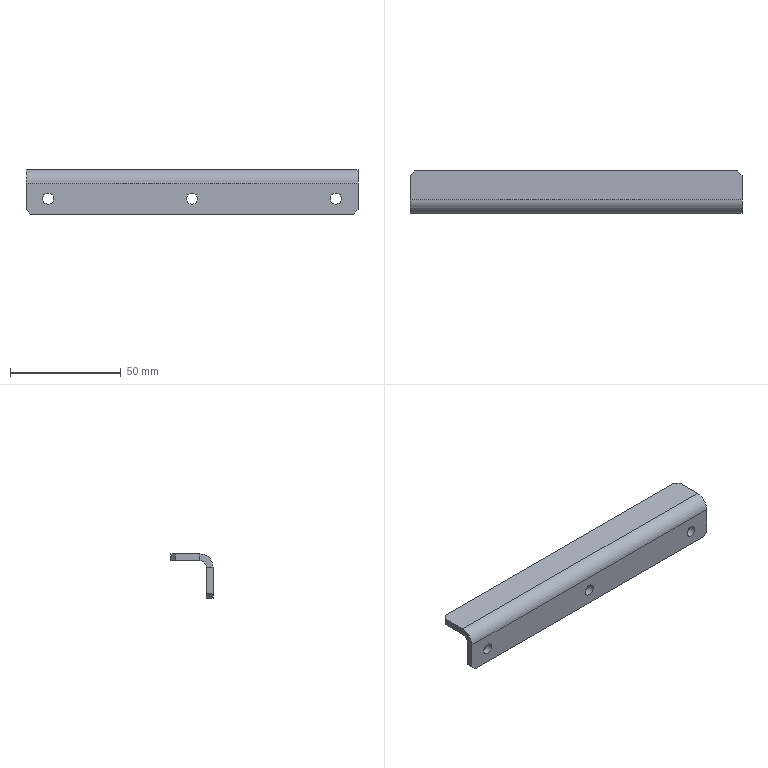Component | SolidWorks | MTCTV2104DJ006-000-0002PressurePlate-1 | 1 solid | 24 faces | box 150 x 19 x 20 mm | volume 15130 mm3 | plane 16 | cylinder 8 | commonest cylinder face diameters 5 x6 12 x1 6 x1
STEP:
#1=CARTESIAN_POINT('',(-7.285,3.002,8.574));
#2=VERTEX_POINT('',#1);
#3=CARTESIAN_POINT('',(-7.482,3.002,8.574));
#4=VERTEX_POINT('',#3);
#5=CARTESIAN_POINT('',(-7.383,3.002,8.574));
#6=DIRECTION('',(-0.,1.,0.));
#7=DIRECTION('',(-1.,0.,0.));
#8=AXIS2_PLACEMENT_3D('',#5,#6,#7);
#9=CIRCLE('',#8,0.09843);
#10=EDGE_CURVE('',#2,#4,#9,.T.);
#11=ORIENTED_EDGE('',*,*,#10,.T.);
#12=CARTESIAN_POINT('',(-7.482,2.884,8.574));
#13=VERTEX_POINT('',#12);
#14=CARTESIAN_POINT('',(-7.482,2.884,8.574));
#15=DIRECTION('',(0.,-1.,-0.));
#16=VECTOR('',#15,39.37);
#17=LINE('',#14,#16);
#18=EDGE_CURVE('',#4,#13,#17,.T.);
#19=ORIENTED_EDGE('',*,*,#18,.T.);
#20=CARTESIAN_POINT('',(-7.285,2.884,8.574));
#21=VERTEX_POINT('',#20);
#22=CARTESIAN_POINT('',(-7.383,2.884,8.574));
#23=DIRECTION('',(0.,-1.,-0.));
#24=DIRECTION('',(1.,0.,0.));
#25=AXIS2_PLACEMENT_3D('',#22,#23,#24);
#26=CIRCLE('',#25,0.09843);
#27=EDGE_CURVE('',#13,#21,#26,.T.);
#28=ORIENTED_EDGE('',*,*,#27,.T.);
#29=CARTESIAN_POINT('',(-7.285,2.884,8.574));
#30=DIRECTION('',(0.,-1.,-0.));
#31=VECTOR('',#30,39.37);
#32=LINE('',#29,#31);
#33=EDGE_CURVE('',#2,#21,#32,.T.);
#34=ORIENTED_EDGE('',*,*,#33,.F.);
#35=EDGE_LOOP('',(#11,#19,#28,#34));
#36=FACE_OUTER_BOUND('',#35,.T.);
#37=CARTESIAN_POINT('',(-7.383,2.884,8.574));
#38=DIRECTION('',(0.,-1.,-0.));
#39=DIRECTION('',(1.,0.,0.));
#40=AXIS2_PLACEMENT_3D('',#37,#38,#39);
#41=CYLINDRICAL_SURFACE('',#40,0.09843);
#42=ADVANCED_FACE('',(#36),#41,.F.);
#43=CARTESIAN_POINT('',(-4.726,3.002,8.574));
#44=VERTEX_POINT('',#43);
#45=CARTESIAN_POINT('',(-4.923,3.002,8.574));
#46=VERTEX_POINT('',#45);
#47=CARTESIAN_POINT('',(-4.824,3.002,8.574));
#48=DIRECTION('',(-0.,1.,0.));
#49=DIRECTION('',(-1.,0.,0.));
#50=AXIS2_PLACEMENT_3D('',#47,#48,#49);
#51=CIRCLE('',#50,0.09843);
#52=EDGE_CURVE('',#44,#46,#51,.T.);
#53=ORIENTED_EDGE('',*,*,#52,.T.);
#54=CARTESIAN_POINT('',(-4.923,2.884,8.574));
#55=VERTEX_POINT('',#54);
#56=CARTESIAN_POINT('',(-4.923,2.884,8.574));
#57=DIRECTION('',(0.,-1.,-0.));
#58=VECTOR('',#57,39.37);
#59=LINE('',#56,#58);
#60=EDGE_CURVE('',#46,#55,#59,.T.);
#61=ORIENTED_EDGE('',*,*,#60,.T.);
#62=CARTESIAN_POINT('',(-4.726,2.884,8.574));
#63=VERTEX_POINT('',#62);
#64=CARTESIAN_POINT('',(-4.824,2.884,8.574));
#65=DIRECTION('',(0.,-1.,-0.));
#66=DIRECTION('',(1.,0.,0.));
#67=AXIS2_PLACEMENT_3D('',#64,#65,#66);
#68=CIRCLE('',#67,0.09843);
#69=EDGE_CURVE('',#55,#63,#68,.T.);
#70=ORIENTED_EDGE('',*,*,#69,.T.);
#71=CARTESIAN_POINT('',(-4.726,2.884,8.574));
#72=DIRECTION('',(0.,-1.,-0.));
#73=VECTOR('',#72,39.37);
#74=LINE('',#71,#73);
#75=EDGE_CURVE('',#44,#63,#74,.T.);
#76=ORIENTED_EDGE('',*,*,#75,.F.);
#77=EDGE_LOOP('',(#53,#61,#70,#76));
#78=FACE_OUTER_BOUND('',#77,.T.);
#79=CARTESIAN_POINT('',(-4.824,2.884,8.574));
#80=DIRECTION('',(0.,-1.,-0.));
#81=DIRECTION('',(1.,0.,0.));
#82=AXIS2_PLACEMENT_3D('',#79,#80,#81);
#83=CYLINDRICAL_SURFACE('',#82,0.09843);
#84=ADVANCED_FACE('',(#78),#83,.F.);
#85=CARTESIAN_POINT('',(-2.167,3.002,8.574));
#86=VERTEX_POINT('',#85);
#87=CARTESIAN_POINT('',(-2.364,3.002,8.574));
#88=VERTEX_POINT('',#87);
#89=CARTESIAN_POINT('',(-2.265,3.002,8.574));
#90=DIRECTION('',(-0.,1.,0.));
#91=DIRECTION('',(-1.,0.,0.));
#92=AXIS2_PLACEMENT_3D('',#89,#90,#91);
#93=CIRCLE('',#92,0.09843);
#94=EDGE_CURVE('',#86,#88,#93,.T.);
#95=ORIENTED_EDGE('',*,*,#94,.T.);
#96=CARTESIAN_POINT('',(-2.364,2.884,8.574));
#97=VERTEX_POINT('',#96);
#98=CARTESIAN_POINT('',(-2.364,2.884,8.574));
#99=DIRECTION('',(0.,-1.,-0.));
#100=VECTOR('',#99,39.37);
#101=LINE('',#98,#100);
#102=EDGE_CURVE('',#88,#97,#101,.T.);
#103=ORIENTED_EDGE('',*,*,#102,.T.);
#104=CARTESIAN_POINT('',(-2.167,2.884,8.574));
#105=VERTEX_POINT('',#104);
#106=CARTESIAN_POINT('',(-2.265,2.884,8.574));
#107=DIRECTION('',(0.,-1.,-0.));
#108=DIRECTION('',(1.,0.,0.));
#109=AXIS2_PLACEMENT_3D('',#106,#107,#108);
#110=CIRCLE('',#109,0.09843);
#111=EDGE_CURVE('',#97,#105,#110,.T.);
#112=ORIENTED_EDGE('',*,*,#111,.T.);
#113=CARTESIAN_POINT('',(-2.167,2.884,8.574));
#114=DIRECTION('',(0.,-1.,-0.));
#115=VECTOR('',#114,39.37);
#116=LINE('',#113,#115);
#117=EDGE_CURVE('',#86,#105,#116,.T.);
#118=ORIENTED_EDGE('',*,*,#117,.F.);
#119=EDGE_LOOP('',(#95,#103,#112,#118));
#120=FACE_OUTER_BOUND('',#119,.T.);
#121=CARTESIAN_POINT('',(-2.265,2.884,8.574));
#122=DIRECTION('',(0.,-1.,-0.));
#123=DIRECTION('',(1.,0.,0.));
#124=AXIS2_PLACEMENT_3D('',#121,#122,#123);
#125=CYLINDRICAL_SURFACE('',#124,0.09843);
#126=ADVANCED_FACE('',(#120),#125,.F.);
#127=CARTESIAN_POINT('',(-7.383,2.884,8.574));
#128=DIRECTION('',(0.,-1.,-0.));
#129=DIRECTION('',(1.,0.,0.));
#130=AXIS2_PLACEMENT_3D('',#127,#128,#129);
#131=CIRCLE('',#130,0.09843);
#132=EDGE_CURVE('',#21,#13,#131,.T.);
#133=ORIENTED_EDGE('',*,*,#132,.F.);
#134=ORIENTED_EDGE('',*,*,#27,.F.);
#135=EDGE_LOOP('',(#133,#134));
#136=FACE_BOUND('',#135,.T.);
#137=CARTESIAN_POINT('',(-2.265,2.884,8.574));
#138=DIRECTION('',(0.,-1.,-0.));
#139=DIRECTION('',(1.,0.,0.));
#140=AXIS2_PLACEMENT_3D('',#137,#138,#139);
#141=CIRCLE('',#140,0.09843);
#142=EDGE_CURVE('',#105,#97,#141,.T.);
#143=ORIENTED_EDGE('',*,*,#142,.F.);
#144=ORIENTED_EDGE('',*,*,#111,.F.);
#145=EDGE_LOOP('',(#143,#144));
#146=FACE_BOUND('',#145,.T.);
#147=CARTESIAN_POINT('',(-7.777,2.884,8.85));
#148=VERTEX_POINT('',#147);
#149=CARTESIAN_POINT('',(-7.777,2.884,8.377));
#150=VERTEX_POINT('',#149);
#151=CARTESIAN_POINT('',(-7.777,2.884,8.299));
#152=DIRECTION('',(-0.,0.,-1.));
#153=VECTOR('',#152,39.37);
#154=LINE('',#151,#153);
#155=EDGE_CURVE('',#148,#150,#154,.T.);
#156=ORIENTED_EDGE('',*,*,#155,.T.);
#157=CARTESIAN_POINT('',(-7.698,2.884,8.299));
#158=VERTEX_POINT('',#157);
#159=CARTESIAN_POINT('',(-7.777,2.884,8.377));
#160=DIRECTION('',(0.7071,0.,-0.7071));
#161=VECTOR('',#160,39.37);
#162=LINE('',#159,#161);
#163=EDGE_CURVE('',#150,#158,#162,.T.);
#164=ORIENTED_EDGE('',*,*,#163,.T.);
#165=CARTESIAN_POINT('',(-1.95,2.884,8.299));
#166=VERTEX_POINT('',#165);
#167=CARTESIAN_POINT('',(-7.777,2.884,8.299));
#168=DIRECTION('',(1.,0.,0.));
#169=VECTOR('',#168,39.37);
#170=LINE('',#167,#169);
#171=EDGE_CURVE('',#158,#166,#170,.T.);
#172=ORIENTED_EDGE('',*,*,#171,.T.);
#173=CARTESIAN_POINT('',(-1.872,2.884,8.377));
#174=VERTEX_POINT('',#173);
#175=CARTESIAN_POINT('',(-1.95,2.884,8.299));
#176=DIRECTION('',(0.7071,-0.,0.7071));
#177=VECTOR('',#176,39.37);
#178=LINE('',#175,#177);
#179=EDGE_CURVE('',#166,#174,#178,.T.);
#180=ORIENTED_EDGE('',*,*,#179,.T.);
#181=CARTESIAN_POINT('',(-1.872,2.884,8.85));
#182=VERTEX_POINT('',#181);
#183=CARTESIAN_POINT('',(-1.872,2.884,8.299));
#184=DIRECTION('',(0.,-0.,1.));
#185=VECTOR('',#184,39.37);
#186=LINE('',#183,#185);
#187=EDGE_CURVE('',#174,#182,#186,.T.);
#188=ORIENTED_EDGE('',*,*,#187,.T.);
#189=CARTESIAN_POINT('',(-1.872,2.884,8.85));
#190=DIRECTION('',(-1.,-0.,-0.));
#191=VECTOR('',#190,39.37);
#192=LINE('',#189,#191);
#193=EDGE_CURVE('',#182,#148,#192,.T.);
#194=ORIENTED_EDGE('',*,*,#193,.T.);
#195=EDGE_LOOP('',(#156,#164,#172,#180,#188,#194));
#196=FACE_OUTER_BOUND('',#195,.T.);
#197=CARTESIAN_POINT('',(-4.824,2.884,8.574));
#198=DIRECTION('',(0.,-1.,-0.));
#199=DIRECTION('',(1.,0.,0.));
#200=AXIS2_PLACEMENT_3D('',#197,#198,#199);
#201=CIRCLE('',#200,0.09843);
#202=EDGE_CURVE('',#63,#55,#201,.T.);
#203=ORIENTED_EDGE('',*,*,#202,.F.);
#204=ORIENTED_EDGE('',*,*,#69,.F.);
#205=EDGE_LOOP('',(#203,#204));
#206=FACE_BOUND('',#205,.T.);
#207=CARTESIAN_POINT('',(-4.824,2.884,8.692));
#208=DIRECTION('',(-0.,1.,0.));
#209=DIRECTION('',(-1.,-0.,-0.));
#210=AXIS2_PLACEMENT_3D('',#207,#208,#209);
#211=PLANE('',#210);
#212=ADVANCED_FACE('',(#136,#146,#196,#206),#211,.F.);
#213=ORIENTED_EDGE('',*,*,#187,.F.);
#214=CARTESIAN_POINT('',(-1.872,3.002,8.377));
#215=VERTEX_POINT('',#214);
#216=CARTESIAN_POINT('',(-1.872,3.002,8.377));
#217=DIRECTION('',(-0.,1.,0.));
#218=VECTOR('',#217,39.37);
#219=LINE('',#216,#218);
#220=EDGE_CURVE('',#174,#215,#219,.T.);
#221=ORIENTED_EDGE('',*,*,#220,.T.);
#222=CARTESIAN_POINT('',(-1.872,3.002,8.85));
#223=VERTEX_POINT('',#222);
#224=CARTESIAN_POINT('',(-1.872,3.002,8.299));
#225=DIRECTION('',(0.,-0.,1.));
#226=VECTOR('',#225,39.37);
#227=LINE('',#224,#226);
#228=EDGE_CURVE('',#215,#223,#227,.T.);
#229=ORIENTED_EDGE('',*,*,#228,.T.);
#230=CARTESIAN_POINT('',(-1.872,3.002,8.85));
#231=DIRECTION('',(0.,-1.,-0.));
#232=VECTOR('',#231,39.37);
#233=LINE('',#230,#232);
#234=EDGE_CURVE('',#223,#182,#233,.T.);
#235=ORIENTED_EDGE('',*,*,#234,.T.);
#236=EDGE_LOOP('',(#213,#221,#229,#235));
#237=FACE_OUTER_BOUND('',#236,.T.);
#238=CARTESIAN_POINT('',(-1.872,3.002,8.299));
#239=DIRECTION('',(1.,0.,0.));
#240=DIRECTION('',(-0.,1.,0.));
#241=AXIS2_PLACEMENT_3D('',#238,#239,#240);
#242=PLANE('',#241);
#243=ADVANCED_FACE('',(#237),#242,.T.);
#244=ORIENTED_EDGE('',*,*,#10,.F.);
#245=CARTESIAN_POINT('',(-7.383,3.002,8.574));
#246=DIRECTION('',(-0.,1.,0.));
#247=DIRECTION('',(-1.,0.,0.));
#248=AXIS2_PLACEMENT_3D('',#245,#246,#247);
#249=CIRCLE('',#248,0.09843);
#250=EDGE_CURVE('',#4,#2,#249,.T.);
#251=ORIENTED_EDGE('',*,*,#250,.F.);
#252=EDGE_LOOP('',(#244,#251));
#253=FACE_BOUND('',#252,.T.);
#254=ORIENTED_EDGE('',*,*,#52,.F.);
#255=CARTESIAN_POINT('',(-4.824,3.002,8.574));
#256=DIRECTION('',(-0.,1.,0.));
#257=DIRECTION('',(-1.,0.,0.));
#258=AXIS2_PLACEMENT_3D('',#255,#256,#257);
#259=CIRCLE('',#258,0.09843);
#260=EDGE_CURVE('',#46,#44,#259,.T.);
#261=ORIENTED_EDGE('',*,*,#260,.F.);
#262=EDGE_LOOP('',(#254,#261));
#263=FACE_BOUND('',#262,.T.);
#264=ORIENTED_EDGE('',*,*,#94,.F.);
#265=CARTESIAN_POINT('',(-2.265,3.002,8.574));
#266=DIRECTION('',(-0.,1.,0.));
#267=DIRECTION('',(-1.,0.,0.));
#268=AXIS2_PLACEMENT_3D('',#265,#266,#267);
#269=CIRCLE('',#268,0.09843);
#270=EDGE_CURVE('',#88,#86,#269,.T.);
#271=ORIENTED_EDGE('',*,*,#270,.F.);
#272=EDGE_LOOP('',(#264,#271));
#273=FACE_BOUND('',#272,.T.);
#274=CARTESIAN_POINT('',(-7.698,3.002,8.299));
#275=VERTEX_POINT('',#274);
#276=CARTESIAN_POINT('',(-1.95,3.002,8.299));
#277=VERTEX_POINT('',#276);
#278=CARTESIAN_POINT('',(-7.777,3.002,8.299));
#279=DIRECTION('',(1.,0.,0.));
#280=VECTOR('',#279,39.37);
#281=LINE('',#278,#280);
#282=EDGE_CURVE('',#275,#277,#281,.T.);
#283=ORIENTED_EDGE('',*,*,#282,.F.);
#284=CARTESIAN_POINT('',(-7.777,3.002,8.377));
#285=VERTEX_POINT('',#284);
#286=CARTESIAN_POINT('',(-6.458,3.002,7.059));
#287=DIRECTION('',(-0.7071,-0.,0.7071));
#288=VECTOR('',#287,39.37);
#289=LINE('',#286,#288);
#290=EDGE_CURVE('',#275,#285,#289,.T.);
#291=ORIENTED_EDGE('',*,*,#290,.T.);
#292=CARTESIAN_POINT('',(-7.777,3.002,8.85));
#293=VERTEX_POINT('',#292);
#294=CARTESIAN_POINT('',(-7.777,3.002,8.299));
#295=DIRECTION('',(-0.,0.,-1.));
#296=VECTOR('',#295,39.37);
#297=LINE('',#294,#296);
#298=EDGE_CURVE('',#293,#285,#297,.T.);
#299=ORIENTED_EDGE('',*,*,#298,.F.);
#300=CARTESIAN_POINT('',(-1.872,3.002,8.85));
#301=DIRECTION('',(-1.,-0.,-0.));
#302=VECTOR('',#301,39.37);
#303=LINE('',#300,#302);
#304=EDGE_CURVE('',#223,#293,#303,.T.);
#305=ORIENTED_EDGE('',*,*,#304,.F.);
#306=ORIENTED_EDGE('',*,*,#228,.F.);
#307=CARTESIAN_POINT('',(-3.19,3.002,7.059));
#308=DIRECTION('',(-0.7071,0.,-0.7071));
#309=VECTOR('',#308,39.37);
#310=LINE('',#307,#309);
#311=EDGE_CURVE('',#215,#277,#310,.T.);
#312=ORIENTED_EDGE('',*,*,#311,.T.);
#313=EDGE_LOOP('',(#283,#291,#299,#305,#306,#312));
#314=FACE_OUTER_BOUND('',#313,.T.);
#315=CARTESIAN_POINT('',(-4.824,3.002,8.692));
#316=DIRECTION('',(-0.,1.,0.));
#317=DIRECTION('',(-1.,-0.,-0.));
#318=AXIS2_PLACEMENT_3D('',#315,#316,#317);
#319=PLANE('',#318);
#320=ADVANCED_FACE('',(#253,#263,#273,#314),#319,.T.);
#321=ORIENTED_EDGE('',*,*,#171,.F.);
#322=CARTESIAN_POINT('',(-7.698,3.002,8.299));
#323=DIRECTION('',(-0.,1.,0.));
#324=VECTOR('',#323,39.37);
#325=LINE('',#322,#324);
#326=EDGE_CURVE('',#158,#275,#325,.T.);
#327=ORIENTED_EDGE('',*,*,#326,.T.);
#328=ORIENTED_EDGE('',*,*,#282,.T.);
#329=CARTESIAN_POINT('',(-1.95,3.002,8.299));
#330=DIRECTION('',(0.,-1.,-0.));
#331=VECTOR('',#330,39.37);
#332=LINE('',#329,#331);
#333=EDGE_CURVE('',#277,#166,#332,.T.);
#334=ORIENTED_EDGE('',*,*,#333,.T.);
#335=EDGE_LOOP('',(#321,#327,#328,#334));
#336=FACE_OUTER_BOUND('',#335,.T.);
#337=CARTESIAN_POINT('',(-7.777,3.002,8.299));
#338=DIRECTION('',(0.,0.,-1.));
#339=DIRECTION('',(1.,0.,0.));
#340=AXIS2_PLACEMENT_3D('',#337,#338,#339);
#341=PLANE('',#340);
#342=ADVANCED_FACE('',(#336),#341,.T.);
#343=ORIENTED_EDGE('',*,*,#298,.T.);
#344=CARTESIAN_POINT('',(-7.777,3.002,8.377));
#345=DIRECTION('',(0.,-1.,-0.));
#346=VECTOR('',#345,39.37);
#347=LINE('',#344,#346);
#348=EDGE_CURVE('',#285,#150,#347,.T.);
#349=ORIENTED_EDGE('',*,*,#348,.T.);
#350=ORIENTED_EDGE('',*,*,#155,.F.);
#351=CARTESIAN_POINT('',(-7.777,3.002,8.85));
#352=DIRECTION('',(0.,-1.,-0.));
#353=VECTOR('',#352,39.37);
#354=LINE('',#351,#353);
#355=EDGE_CURVE('',#293,#148,#354,.T.);
#356=ORIENTED_EDGE('',*,*,#355,.F.);
#357=EDGE_LOOP('',(#343,#349,#350,#356));
#358=FACE_OUTER_BOUND('',#357,.T.);
#359=CARTESIAN_POINT('',(-7.777,3.002,8.299));
#360=DIRECTION('',(-1.,-0.,-0.));
#361=DIRECTION('',(0.,-1.,-0.));
#362=AXIS2_PLACEMENT_3D('',#359,#360,#361);
#363=PLANE('',#362);
#364=ADVANCED_FACE('',(#358),#363,.T.);
#365=CARTESIAN_POINT('',(-7.777,3.12,8.968));
#366=VERTEX_POINT('',#365);
#367=CARTESIAN_POINT('',(-7.777,3.12,9.086));
#368=VERTEX_POINT('',#367);
#369=CARTESIAN_POINT('',(-7.777,3.12,9.086));
#370=DIRECTION('',(0.,-0.,1.));
#371=VECTOR('',#370,39.37);
#372=LINE('',#369,#371);
#373=EDGE_CURVE('',#366,#368,#372,.T.);
#374=ORIENTED_EDGE('',*,*,#373,.F.);
#375=CARTESIAN_POINT('',(-7.777,3.12,8.85));
#376=DIRECTION('',(-1.,-0.,-0.));
#377=DIRECTION('',(0.,1.,0.));
#378=AXIS2_PLACEMENT_3D('',#375,#376,#377);
#379=CIRCLE('',#378,0.1181);
#380=EDGE_CURVE('',#293,#366,#379,.T.);
#381=ORIENTED_EDGE('',*,*,#380,.F.);
#382=ORIENTED_EDGE('',*,*,#355,.T.);
#383=CARTESIAN_POINT('',(-7.777,3.12,8.85));
#384=DIRECTION('',(-1.,-0.,-0.));
#385=DIRECTION('',(0.,1.,0.));
#386=AXIS2_PLACEMENT_3D('',#383,#384,#385);
#387=CIRCLE('',#386,0.2362);
#388=EDGE_CURVE('',#148,#368,#387,.T.);
#389=ORIENTED_EDGE('',*,*,#388,.T.);
#390=EDGE_LOOP('',(#374,#381,#382,#389));
#391=FACE_OUTER_BOUND('',#390,.T.);
#392=CARTESIAN_POINT('',(-7.777,3.12,8.85));
#393=DIRECTION('',(-1.,-0.,-0.));
#394=DIRECTION('',(0.,-1.,-0.));
#395=AXIS2_PLACEMENT_3D('',#392,#393,#394);
#396=PLANE('',#395);
#397=ADVANCED_FACE('',(#391),#396,.T.);
#398=CARTESIAN_POINT('',(-1.872,3.12,8.968));
#399=VERTEX_POINT('',#398);
#400=CARTESIAN_POINT('',(-1.872,3.12,8.85));
#401=DIRECTION('',(1.,0.,0.));
#402=DIRECTION('',(0.,1.,0.));
#403=AXIS2_PLACEMENT_3D('',#400,#401,#402);
#404=CIRCLE('',#403,0.1181);
#405=EDGE_CURVE('',#399,#223,#404,.T.);
#406=ORIENTED_EDGE('',*,*,#405,.F.);
#407=CARTESIAN_POINT('',(-1.872,3.12,9.086));
#408=VERTEX_POINT('',#407);
#409=CARTESIAN_POINT('',(-1.872,3.12,8.968));
#410=DIRECTION('',(0.,-0.,1.));
#411=VECTOR('',#410,39.37);
#412=LINE('',#409,#411);
#413=EDGE_CURVE('',#399,#408,#412,.T.);
#414=ORIENTED_EDGE('',*,*,#413,.T.);
#415=CARTESIAN_POINT('',(-1.872,3.12,8.85));
#416=DIRECTION('',(1.,0.,0.));
#417=DIRECTION('',(0.,1.,0.));
#418=AXIS2_PLACEMENT_3D('',#415,#416,#417);
#419=CIRCLE('',#418,0.2362);
#420=EDGE_CURVE('',#408,#182,#419,.T.);
#421=ORIENTED_EDGE('',*,*,#420,.T.);
#422=ORIENTED_EDGE('',*,*,#234,.F.);
#423=EDGE_LOOP('',(#406,#414,#421,#422));
#424=FACE_OUTER_BOUND('',#423,.T.);
#425=CARTESIAN_POINT('',(-1.872,3.12,8.85));
#426=DIRECTION('',(-1.,-0.,-0.));
#427=DIRECTION('',(0.,-1.,-0.));
#428=AXIS2_PLACEMENT_3D('',#425,#426,#427);
#429=PLANE('',#428);
#430=ADVANCED_FACE('',(#424),#429,.F.);
#431=ORIENTED_EDGE('',*,*,#193,.F.);
#432=ORIENTED_EDGE('',*,*,#420,.F.);
#433=CARTESIAN_POINT('',(-7.777,3.12,9.086));
#434=DIRECTION('',(-1.,-0.,-0.));
#435=VECTOR('',#434,39.37);
#436=LINE('',#433,#435);
#437=EDGE_CURVE('',#408,#368,#436,.T.);
#438=ORIENTED_EDGE('',*,*,#437,.T.);
#439=ORIENTED_EDGE('',*,*,#388,.F.);
#440=EDGE_LOOP('',(#431,#432,#438,#439));
#441=FACE_OUTER_BOUND('',#440,.T.);
#442=CARTESIAN_POINT('',(-1.872,3.12,8.85));
#443=DIRECTION('',(1.,0.,0.));
#444=DIRECTION('',(0.,-0.,1.));
#445=AXIS2_PLACEMENT_3D('',#442,#443,#444);
#446=CYLINDRICAL_SURFACE('',#445,0.2362);
#447=ADVANCED_FACE('',(#441),#446,.T.);
#448=ORIENTED_EDGE('',*,*,#304,.T.);
#449=ORIENTED_EDGE('',*,*,#380,.T.);
#450=CARTESIAN_POINT('',(-7.777,3.12,8.968));
#451=DIRECTION('',(1.,0.,0.));
#452=VECTOR('',#451,39.37);
#453=LINE('',#450,#452);
#454=EDGE_CURVE('',#366,#399,#453,.T.);
#455=ORIENTED_EDGE('',*,*,#454,.T.);
#456=ORIENTED_EDGE('',*,*,#405,.T.);
#457=EDGE_LOOP('',(#448,#449,#455,#456));
#458=FACE_OUTER_BOUND('',#457,.T.);
#459=CARTESIAN_POINT('',(-1.872,3.12,8.85));
#460=DIRECTION('',(1.,0.,0.));
#461=DIRECTION('',(0.,-0.,1.));
#462=AXIS2_PLACEMENT_3D('',#459,#460,#461);
#463=CYLINDRICAL_SURFACE('',#462,0.1181);
#464=ADVANCED_FACE('',(#458),#463,.F.);
#465=CARTESIAN_POINT('',(-1.872,3.553,8.968));
#466=VERTEX_POINT('',#465);
#467=CARTESIAN_POINT('',(-1.872,3.632,8.968));
#468=DIRECTION('',(-0.,1.,0.));
#469=VECTOR('',#468,39.37);
#470=LINE('',#467,#469);
#471=EDGE_CURVE('',#399,#466,#470,.T.);
#472=ORIENTED_EDGE('',*,*,#471,.T.);
#473=CARTESIAN_POINT('',(-1.872,3.553,9.086));
#474=VERTEX_POINT('',#473);
#475=CARTESIAN_POINT('',(-1.872,3.553,9.086));
#476=DIRECTION('',(0.,-0.,1.));
#477=VECTOR('',#476,39.37);
#478=LINE('',#475,#477);
#479=EDGE_CURVE('',#466,#474,#478,.T.);
#480=ORIENTED_EDGE('',*,*,#479,.T.);
#481=CARTESIAN_POINT('',(-1.872,2.884,9.086));
#482=DIRECTION('',(-0.,1.,0.));
#483=VECTOR('',#482,39.37);
#484=LINE('',#481,#483);
#485=EDGE_CURVE('',#408,#474,#484,.T.);
#486=ORIENTED_EDGE('',*,*,#485,.F.);
#487=ORIENTED_EDGE('',*,*,#413,.F.);
#488=EDGE_LOOP('',(#472,#480,#486,#487));
#489=FACE_OUTER_BOUND('',#488,.T.);
#490=CARTESIAN_POINT('',(-1.872,3.632,9.086));
#491=DIRECTION('',(-1.,-0.,-0.));
#492=DIRECTION('',(0.,-1.,-0.));
#493=AXIS2_PLACEMENT_3D('',#490,#491,#492);
#494=PLANE('',#493);
#495=ADVANCED_FACE('',(#489),#494,.F.);
#496=CARTESIAN_POINT('',(-7.777,3.553,9.086));
#497=VERTEX_POINT('',#496);
#498=CARTESIAN_POINT('',(-7.777,2.884,9.086));
#499=DIRECTION('',(0.,-1.,-0.));
#500=VECTOR('',#499,39.37);
#501=LINE('',#498,#500);
#502=EDGE_CURVE('',#497,#368,#501,.T.);
#503=ORIENTED_EDGE('',*,*,#502,.F.);
#504=CARTESIAN_POINT('',(-7.777,3.553,8.968));
#505=VERTEX_POINT('',#504);
#506=CARTESIAN_POINT('',(-7.777,3.553,9.086));
#507=DIRECTION('',(-0.,0.,-1.));
#508=VECTOR('',#507,39.37);
#509=LINE('',#506,#508);
#510=EDGE_CURVE('',#497,#505,#509,.T.);
#511=ORIENTED_EDGE('',*,*,#510,.T.);
#512=CARTESIAN_POINT('',(-7.777,3.002,8.968));
#513=DIRECTION('',(0.,-1.,-0.));
#514=VECTOR('',#513,39.37);
#515=LINE('',#512,#514);
#516=EDGE_CURVE('',#505,#366,#515,.T.);
#517=ORIENTED_EDGE('',*,*,#516,.T.);
#518=ORIENTED_EDGE('',*,*,#373,.T.);
#519=EDGE_LOOP('',(#503,#511,#517,#518));
#520=FACE_OUTER_BOUND('',#519,.T.);
#521=CARTESIAN_POINT('',(-7.777,3.002,9.086));
#522=DIRECTION('',(1.,0.,0.));
#523=DIRECTION('',(-0.,1.,0.));
#524=AXIS2_PLACEMENT_3D('',#521,#522,#523);
#525=PLANE('',#524);
#526=ADVANCED_FACE('',(#520),#525,.F.);
#527=ORIENTED_EDGE('',*,*,#485,.T.);
#528=CARTESIAN_POINT('',(-1.95,3.632,9.086));
#529=VERTEX_POINT('',#528);
#530=CARTESIAN_POINT('',(-1.95,3.632,9.086));
#531=DIRECTION('',(-0.7071,0.7071,0.));
#532=VECTOR('',#531,39.37);
#533=LINE('',#530,#532);
#534=EDGE_CURVE('',#474,#529,#533,.T.);
#535=ORIENTED_EDGE('',*,*,#534,.T.);
#536=CARTESIAN_POINT('',(-7.698,3.632,9.086));
#537=VERTEX_POINT('',#536);
#538=CARTESIAN_POINT('',(-4.824,3.632,9.086));
#539=DIRECTION('',(-1.,-0.,-0.));
#540=VECTOR('',#539,39.37);
#541=LINE('',#538,#540);
#542=EDGE_CURVE('',#529,#537,#541,.T.);
#543=ORIENTED_EDGE('',*,*,#542,.T.);
#544=CARTESIAN_POINT('',(-7.777,3.553,9.086));
#545=DIRECTION('',(-0.7071,-0.7071,-0.));
#546=VECTOR('',#545,39.37);
#547=LINE('',#544,#546);
#548=EDGE_CURVE('',#537,#497,#547,.T.);
#549=ORIENTED_EDGE('',*,*,#548,.T.);
#550=ORIENTED_EDGE('',*,*,#502,.T.);
#551=ORIENTED_EDGE('',*,*,#437,.F.);
#552=EDGE_LOOP('',(#527,#535,#543,#549,#550,#551));
#553=FACE_OUTER_BOUND('',#552,.T.);
#554=CARTESIAN_POINT('',(-4.824,2.884,9.086));
#555=DIRECTION('',(-0.,0.,-1.));
#556=DIRECTION('',(0.,-1.,-0.));
#557=AXIS2_PLACEMENT_3D('',#554,#555,#556);
#558=PLANE('',#557);
#559=ADVANCED_FACE('',(#553),#558,.F.);
#560=CARTESIAN_POINT('',(-1.95,3.632,8.968));
#561=VERTEX_POINT('',#560);
#562=CARTESIAN_POINT('',(-7.698,3.632,8.968));
#563=VERTEX_POINT('',#562);
#564=CARTESIAN_POINT('',(-7.777,3.632,8.968));
#565=DIRECTION('',(-1.,-0.,-0.));
#566=VECTOR('',#565,39.37);
#567=LINE('',#564,#566);
#568=EDGE_CURVE('',#561,#563,#567,.T.);
#569=ORIENTED_EDGE('',*,*,#568,.F.);
#570=CARTESIAN_POINT('',(-3.013,4.695,8.968));
#571=DIRECTION('',(0.7071,-0.7071,-0.));
#572=VECTOR('',#571,39.37);
#573=LINE('',#570,#572);
#574=EDGE_CURVE('',#561,#466,#573,.T.);
#575=ORIENTED_EDGE('',*,*,#574,.T.);
#576=ORIENTED_EDGE('',*,*,#471,.F.);
#577=ORIENTED_EDGE('',*,*,#454,.F.);
#578=ORIENTED_EDGE('',*,*,#516,.F.);
#579=CARTESIAN_POINT('',(-6.635,4.695,8.968));
#580=DIRECTION('',(0.7071,0.7071,0.));
#581=VECTOR('',#580,39.37);
#582=LINE('',#579,#581);
#583=EDGE_CURVE('',#505,#563,#582,.T.);
#584=ORIENTED_EDGE('',*,*,#583,.T.);
#585=EDGE_LOOP('',(#569,#575,#576,#577,#578,#584));
#586=FACE_OUTER_BOUND('',#585,.T.);
#587=CARTESIAN_POINT('',(-4.824,2.884,8.968));
#588=DIRECTION('',(-0.,0.,-1.));
#589=DIRECTION('',(0.,-1.,-0.));
#590=AXIS2_PLACEMENT_3D('',#587,#588,#589);
#591=PLANE('',#590);
#592=ADVANCED_FACE('',(#586),#591,.T.);
#593=ORIENTED_EDGE('',*,*,#542,.F.);
#594=CARTESIAN_POINT('',(-1.95,3.632,9.086));
#595=DIRECTION('',(-0.,0.,-1.));
#596=VECTOR('',#595,39.37);
#597=LINE('',#594,#596);
#598=EDGE_CURVE('',#529,#561,#597,.T.);
#599=ORIENTED_EDGE('',*,*,#598,.T.);
#600=ORIENTED_EDGE('',*,*,#568,.T.);
#601=CARTESIAN_POINT('',(-7.698,3.632,9.086));
#602=DIRECTION('',(0.,-0.,1.));
#603=VECTOR('',#602,39.37);
#604=LINE('',#601,#603);
#605=EDGE_CURVE('',#563,#537,#604,.T.);
#606=ORIENTED_EDGE('',*,*,#605,.T.);
#607=EDGE_LOOP('',(#593,#599,#600,#606));
#608=FACE_OUTER_BOUND('',#607,.T.);
#609=CARTESIAN_POINT('',(-7.777,3.632,9.086));
#610=DIRECTION('',(0.,-1.,-0.));
#611=DIRECTION('',(0.,-0.,1.));
#612=AXIS2_PLACEMENT_3D('',#609,#610,#611);
#613=PLANE('',#612);
#614=ADVANCED_FACE('',(#608),#613,.F.);
#615=ORIENTED_EDGE('',*,*,#102,.F.);
#616=ORIENTED_EDGE('',*,*,#270,.T.);
#617=ORIENTED_EDGE('',*,*,#117,.T.);
#618=ORIENTED_EDGE('',*,*,#142,.T.);
#619=EDGE_LOOP('',(#615,#616,#617,#618));
#620=FACE_OUTER_BOUND('',#619,.T.);
#621=CARTESIAN_POINT('',(-2.265,2.884,8.574));
#622=DIRECTION('',(0.,-1.,-0.));
#623=DIRECTION('',(1.,0.,0.));
#624=AXIS2_PLACEMENT_3D('',#621,#622,#623);
#625=CYLINDRICAL_SURFACE('',#624,0.09843);
#626=ADVANCED_FACE('',(#620),#625,.F.);
#627=ORIENTED_EDGE('',*,*,#60,.F.);
#628=ORIENTED_EDGE('',*,*,#260,.T.);
#629=ORIENTED_EDGE('',*,*,#75,.T.);
#630=ORIENTED_EDGE('',*,*,#202,.T.);
#631=EDGE_LOOP('',(#627,#628,#629,#630));
#632=FACE_OUTER_BOUND('',#631,.T.);
#633=CARTESIAN_POINT('',(-4.824,2.884,8.574));
#634=DIRECTION('',(0.,-1.,-0.));
#635=DIRECTION('',(1.,0.,0.));
#636=AXIS2_PLACEMENT_3D('',#633,#634,#635);
#637=CYLINDRICAL_SURFACE('',#636,0.09843);
#638=ADVANCED_FACE('',(#632),#637,.F.);
#639=ORIENTED_EDGE('',*,*,#18,.F.);
#640=ORIENTED_EDGE('',*,*,#250,.T.);
#641=ORIENTED_EDGE('',*,*,#33,.T.);
#642=ORIENTED_EDGE('',*,*,#132,.T.);
#643=EDGE_LOOP('',(#639,#640,#641,#642));
#644=FACE_OUTER_BOUND('',#643,.T.);
#645=CARTESIAN_POINT('',(-7.383,2.884,8.574));
#646=DIRECTION('',(0.,-1.,-0.));
#647=DIRECTION('',(1.,0.,0.));
#648=AXIS2_PLACEMENT_3D('',#645,#646,#647);
#649=CYLINDRICAL_SURFACE('',#648,0.09843);
#650=ADVANCED_FACE('',(#644),#649,.F.);
#651=ORIENTED_EDGE('',*,*,#290,.F.);
#652=ORIENTED_EDGE('',*,*,#326,.F.);
#653=ORIENTED_EDGE('',*,*,#163,.F.);
#654=ORIENTED_EDGE('',*,*,#348,.F.);
#655=EDGE_LOOP('',(#651,#652,#653,#654));
#656=FACE_OUTER_BOUND('',#655,.T.);
#657=CARTESIAN_POINT('',(-7.777,3.002,8.377));
#658=DIRECTION('',(0.7071,-0.,0.7071));
#659=DIRECTION('',(0.,-1.,-0.));
#660=AXIS2_PLACEMENT_3D('',#657,#658,#659);
#661=PLANE('',#660);
#662=ADVANCED_FACE('',(#656),#661,.F.);
#663=ORIENTED_EDGE('',*,*,#311,.F.);
#664=ORIENTED_EDGE('',*,*,#220,.F.);
#665=ORIENTED_EDGE('',*,*,#179,.F.);
#666=ORIENTED_EDGE('',*,*,#333,.F.);
#667=EDGE_LOOP('',(#663,#664,#665,#666));
#668=FACE_OUTER_BOUND('',#667,.T.);
#669=CARTESIAN_POINT('',(-1.95,3.002,8.299));
#670=DIRECTION('',(-0.7071,-0.,0.7071));
#671=DIRECTION('',(0.,-1.,-0.));
#672=AXIS2_PLACEMENT_3D('',#669,#670,#671);
#673=PLANE('',#672);
#674=ADVANCED_FACE('',(#668),#673,.F.);
#675=ORIENTED_EDGE('',*,*,#534,.F.);
#676=ORIENTED_EDGE('',*,*,#479,.F.);
#677=ORIENTED_EDGE('',*,*,#574,.F.);
#678=ORIENTED_EDGE('',*,*,#598,.F.);
#679=EDGE_LOOP('',(#675,#676,#677,#678));
#680=FACE_OUTER_BOUND('',#679,.T.);
#681=CARTESIAN_POINT('',(-1.95,3.632,9.086));
#682=DIRECTION('',(-0.7071,-0.7071,-0.));
#683=DIRECTION('',(-0.,0.,-1.));
#684=AXIS2_PLACEMENT_3D('',#681,#682,#683);
#685=PLANE('',#684);
#686=ADVANCED_FACE('',(#680),#685,.F.);
#687=ORIENTED_EDGE('',*,*,#548,.F.);
#688=ORIENTED_EDGE('',*,*,#605,.F.);
#689=ORIENTED_EDGE('',*,*,#583,.F.);
#690=ORIENTED_EDGE('',*,*,#510,.F.);
#691=EDGE_LOOP('',(#687,#688,#689,#690));
#692=FACE_OUTER_BOUND('',#691,.T.);
#693=CARTESIAN_POINT('',(-7.777,3.553,9.086));
#694=DIRECTION('',(0.7071,-0.7071,-0.));
#695=DIRECTION('',(-0.,0.,-1.));
#696=AXIS2_PLACEMENT_3D('',#693,#694,#695);
#697=PLANE('',#696);
#698=ADVANCED_FACE('',(#692),#697,.F.);
#699=CLOSED_SHELL('',(#42,#84,#126,#212,#243,#320,#342,#364,#397,#430,#447,#464,#495,#526,#559,#592,#614,#626,#638,#650,#662,#674,#686,#698));
#700=MANIFOLD_SOLID_BREP('',#699);
#701=CARTESIAN_POINT('',(0.,0.,0.));
#702=DIRECTION('',(0.,0.,1.));
#703=DIRECTION('',(1.,0.,0.));
#704=AXIS2_PLACEMENT_3D('',#701,#702,#703);
#705=(LENGTH_UNIT()NAMED_UNIT(*)SI_UNIT($,.METRE.));
#706=LENGTH_MEASURE_WITH_UNIT(LENGTH_MEASURE(0.0254),#705);
#707=DIMENSIONAL_EXPONENTS(1.,0.,0.,0.,0.,0.,0.);
#708=(CONVERSION_BASED_UNIT('',#706)LENGTH_UNIT()NAMED_UNIT(#707));
#709=UNCERTAINTY_MEASURE_WITH_UNIT(LENGTH_MEASURE(0.00001),#708,'','');
#710=(NAMED_UNIT(*)PLANE_ANGLE_UNIT()SI_UNIT($,.RADIAN.));
#711=(NAMED_UNIT(*)SI_UNIT($,.STERADIAN.)SOLID_ANGLE_UNIT());
#712=(GEOMETRIC_REPRESENTATION_CONTEXT(3)GLOBAL_UNCERTAINTY_ASSIGNED_CONTEXT((#709))GLOBAL_UNIT_ASSIGNED_CONTEXT((#708,#710,#711))REPRESENTATION_CONTEXT('',''));
#713=ADVANCED_BREP_SHAPE_REPRESENTATION('',(#700,#704),#712);
#714=COLOUR_RGB('',0.7922,0.8196,0.9333);
#715=FILL_AREA_STYLE_COLOUR('',#714);
#716=FILL_AREA_STYLE('',(#715));
#717=SURFACE_STYLE_FILL_AREA(#716);
#718=SURFACE_SIDE_STYLE('',(#717));
#719=SURFACE_STYLE_USAGE(.BOTH.,#718);
#720=PRESENTATION_STYLE_ASSIGNMENT((#719));
#721=STYLED_ITEM('',(#720),#700);
#722=(LENGTH_UNIT()NAMED_UNIT(*)SI_UNIT($,.METRE.));
#723=LENGTH_MEASURE_WITH_UNIT(LENGTH_MEASURE(0.0254),#722);
#724=DIMENSIONAL_EXPONENTS(1.,0.,0.,0.,0.,0.,0.);
#725=(CONVERSION_BASED_UNIT('',#723)LENGTH_UNIT()NAMED_UNIT(#724));
#726=UNCERTAINTY_MEASURE_WITH_UNIT(LENGTH_MEASURE(0.00001),#725,'','');
#727=(NAMED_UNIT(*)PLANE_ANGLE_UNIT()SI_UNIT($,.RADIAN.));
#728=(NAMED_UNIT(*)SI_UNIT($,.STERADIAN.)SOLID_ANGLE_UNIT());
#729=(GEOMETRIC_REPRESENTATION_CONTEXT(3)GLOBAL_UNCERTAINTY_ASSIGNED_CONTEXT((#726))GLOBAL_UNIT_ASSIGNED_CONTEXT((#725,#727,#728))REPRESENTATION_CONTEXT('',''));
#730=MECHANICAL_DESIGN_GEOMETRIC_PRESENTATION_REPRESENTATION('',(#721),#729);
#731=PRESENTATION_LAYER_ASSIGNMENT('','',(#721));